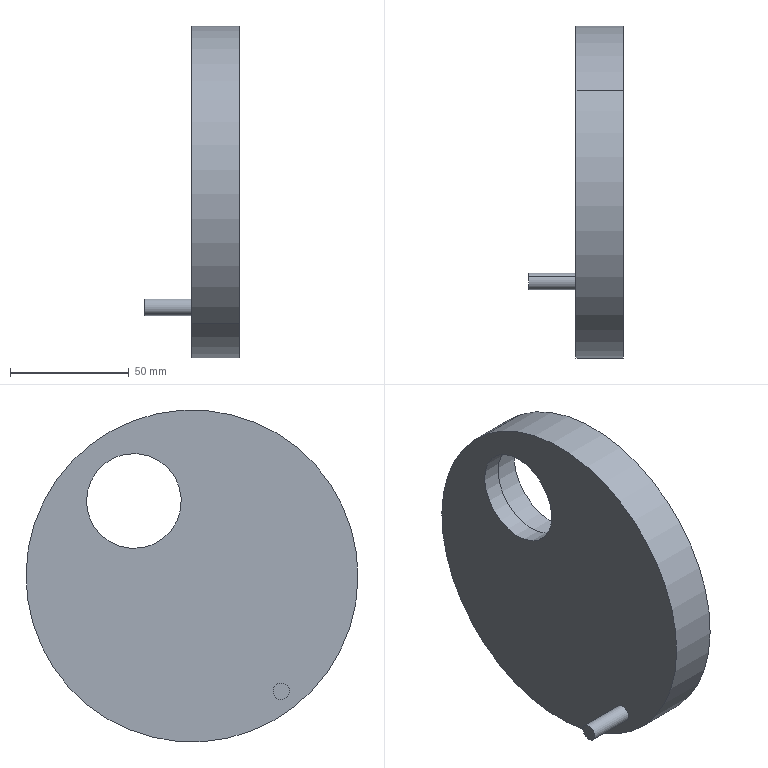Component | SolidWorks | Part1-1 | 1 solid | 12 faces | box 40 x 140 x 140 mm | volume 279507 mm3 | cylinder 8 | plane 4 | commonest cylinder face diameters 45 x2 7 x2 140 x2 40 x2
build123d program:
from build123d import *

# Parameters (mm, degrees)
SKETCH1_2_R          = 70
BOSS_EXTRUDE1_DEPTH  = 20
SKETCH2_R            = 20
CUT_EXTRUDE1_2_DEPTH = 20
SKETCH3_R            = 3.5
BOSS_EXTRUDE2_DEPTH  = 20
SKETCH1_R            = 22.5
CUT_EXTRUDE1_DEPTH   = 12


with BuildPart() as part:
    # Sketch1_2 → Boss-Extrude1 (new body)
    with BuildSketch(Plane(origin=(0, 0, 0), x_dir=(0, 0, -1), z_dir=(1, 0, 0))):
        Circle(SKETCH1_2_R)
    extrude(amount=BOSS_EXTRUDE1_DEPTH)

    # Sketch2 → Cut-Extrude1_2 (cut)
    with BuildSketch(Plane(origin=(20, 0, 0), x_dir=(0, 0, -1), z_dir=(1, 0, 0))):
        with Locations((40, 0)):
            Circle(SKETCH2_R)
    extrude(amount=-CUT_EXTRUDE1_2_DEPTH, mode=Mode.SUBTRACT)

    # Sketch3 → Boss-Extrude2 (add)
    with BuildSketch(Plane(origin=(20, 0, 0), x_dir=(0, 0, -1), z_dir=(1, 0, 0))):
        with Locations((-61.5, 0)):
            Circle(SKETCH3_R)
    extrude(amount=BOSS_EXTRUDE2_DEPTH)

    # Sketch1 → Cut-Extrude1 (cut)
    with BuildSketch(Plane.ZY):
        with Locations((-40, 0)):
            Circle(SKETCH1_R)
    extrude(amount=-CUT_EXTRUDE1_DEPTH, mode=Mode.SUBTRACT)


solid = part.part

# Placed as in the assembly
solid = solid.moved(Location((405.528, -9.187, -141.621), (142.235, 0, -180)))
STEP:
#1=COLOUR_RGB('',0.7922,0.8196,0.9333);
#2=FILL_AREA_STYLE_COLOUR('',#1);
#3=FILL_AREA_STYLE('',(#2));
#4=SURFACE_STYLE_FILL_AREA(#3);
#5=SURFACE_SIDE_STYLE('',(#4));
#6=SURFACE_STYLE_USAGE(.BOTH.,#5);
#7=PRESENTATION_STYLE_ASSIGNMENT((#6));
#8=CARTESIAN_POINT('',(15.493,1.145,-3.63));
#9=VERTEX_POINT('',#8);
#10=CARTESIAN_POINT('',(15.493,0.06026,-5.031));
#11=VERTEX_POINT('',#10);
#12=CARTESIAN_POINT('',(15.493,0.6028,-4.331));
#13=DIRECTION('',(1.,0.,0.));
#14=DIRECTION('',(0.,-0.6124,-0.7905));
#15=AXIS2_PLACEMENT_3D('',#12,#13,#14);
#16=CIRCLE('',#15,0.8858);
#17=EDGE_CURVE('',#9,#11,#16,.T.);
#18=ORIENTED_EDGE('',*,*,#17,.F.);
#19=CARTESIAN_POINT('',(15.966,1.145,-3.63));
#20=VERTEX_POINT('',#19);
#21=CARTESIAN_POINT('',(15.493,1.145,-3.63));
#22=DIRECTION('',(1.,0.,0.));
#23=VECTOR('',#22,39.37);
#24=LINE('',#21,#23);
#25=EDGE_CURVE('',#9,#20,#24,.T.);
#26=ORIENTED_EDGE('',*,*,#25,.T.);
#27=CARTESIAN_POINT('',(15.966,0.06026,-5.031));
#28=VERTEX_POINT('',#27);
#29=CARTESIAN_POINT('',(15.966,0.6028,-4.331));
#30=DIRECTION('',(1.,0.,0.));
#31=DIRECTION('',(0.,-0.6124,-0.7905));
#32=AXIS2_PLACEMENT_3D('',#29,#30,#31);
#33=CIRCLE('',#32,0.8858);
#34=EDGE_CURVE('',#20,#28,#33,.T.);
#35=ORIENTED_EDGE('',*,*,#34,.T.);
#36=CARTESIAN_POINT('',(15.493,0.06026,-5.031));
#37=DIRECTION('',(1.,0.,0.));
#38=VECTOR('',#37,39.37);
#39=LINE('',#36,#38);
#40=EDGE_CURVE('',#11,#28,#39,.T.);
#41=ORIENTED_EDGE('',*,*,#40,.F.);
#42=EDGE_LOOP('',(#18,#26,#35,#41));
#43=FACE_OUTER_BOUND('',#42,.T.);
#44=CARTESIAN_POINT('',(15.493,0.6028,-4.331));
#45=DIRECTION('',(1.,0.,0.));
#46=DIRECTION('',(0.,-0.6124,-0.7905));
#47=AXIS2_PLACEMENT_3D('',#44,#45,#46);
#48=CYLINDRICAL_SURFACE('',#47,0.8858);
#49=ADVANCED_FACE('',(#43),#48,.F.);
#50=CARTESIAN_POINT('',(14.391,-1.76,-7.381));
#51=VERTEX_POINT('',#50);
#52=CARTESIAN_POINT('',(14.391,-1.929,-7.599));
#53=VERTEX_POINT('',#52);
#54=CARTESIAN_POINT('',(14.391,-1.845,-7.49));
#55=DIRECTION('',(-1.,0.,0.));
#56=DIRECTION('',(0.,0.6124,0.7905));
#57=AXIS2_PLACEMENT_3D('',#54,#55,#56);
#58=CIRCLE('',#57,0.1378);
#59=EDGE_CURVE('',#51,#53,#58,.T.);
#60=ORIENTED_EDGE('',*,*,#59,.F.);
#61=CARTESIAN_POINT('',(15.178,-1.76,-7.381));
#62=VERTEX_POINT('',#61);
#63=CARTESIAN_POINT('',(14.391,-1.76,-7.381));
#64=DIRECTION('',(1.,0.,0.));
#65=VECTOR('',#64,39.37);
#66=LINE('',#63,#65);
#67=EDGE_CURVE('',#51,#62,#66,.T.);
#68=ORIENTED_EDGE('',*,*,#67,.T.);
#69=CARTESIAN_POINT('',(15.178,-1.929,-7.599));
#70=VERTEX_POINT('',#69);
#71=CARTESIAN_POINT('',(15.178,-1.845,-7.49));
#72=DIRECTION('',(-1.,0.,0.));
#73=DIRECTION('',(0.,0.6124,0.7905));
#74=AXIS2_PLACEMENT_3D('',#71,#72,#73);
#75=CIRCLE('',#74,0.1378);
#76=EDGE_CURVE('',#62,#70,#75,.T.);
#77=ORIENTED_EDGE('',*,*,#76,.T.);
#78=CARTESIAN_POINT('',(14.391,-1.929,-7.599));
#79=DIRECTION('',(1.,0.,0.));
#80=VECTOR('',#79,39.37);
#81=LINE('',#78,#80);
#82=EDGE_CURVE('',#53,#70,#81,.T.);
#83=ORIENTED_EDGE('',*,*,#82,.F.);
#84=EDGE_LOOP('',(#60,#68,#77,#83));
#85=FACE_OUTER_BOUND('',#84,.T.);
#86=CARTESIAN_POINT('',(14.391,-1.845,-7.49));
#87=DIRECTION('',(1.,0.,0.));
#88=DIRECTION('',(0.,-0.6124,-0.7905));
#89=AXIS2_PLACEMENT_3D('',#86,#87,#88);
#90=CYLINDRICAL_SURFACE('',#89,0.1378);
#91=ADVANCED_FACE('',(#85),#90,.T.);
#92=CARTESIAN_POINT('',(15.178,1.326,-3.397));
#93=VERTEX_POINT('',#92);
#94=CARTESIAN_POINT('',(15.178,-2.049,-7.754));
#95=VERTEX_POINT('',#94);
#96=CARTESIAN_POINT('',(15.178,-0.3617,-5.576));
#97=DIRECTION('',(-1.,0.,0.));
#98=DIRECTION('',(0.,0.6124,0.7905));
#99=AXIS2_PLACEMENT_3D('',#96,#97,#98);
#100=CIRCLE('',#99,2.756);
#101=EDGE_CURVE('',#93,#95,#100,.T.);
#102=ORIENTED_EDGE('',*,*,#101,.F.);
#103=CARTESIAN_POINT('',(15.966,1.326,-3.397));
#104=VERTEX_POINT('',#103);
#105=CARTESIAN_POINT('',(15.178,1.326,-3.397));
#106=DIRECTION('',(1.,0.,0.));
#107=VECTOR('',#106,39.37);
#108=LINE('',#105,#107);
#109=EDGE_CURVE('',#93,#104,#108,.T.);
#110=ORIENTED_EDGE('',*,*,#109,.T.);
#111=CARTESIAN_POINT('',(15.966,-2.049,-7.754));
#112=VERTEX_POINT('',#111);
#113=CARTESIAN_POINT('',(15.966,-0.3617,-5.576));
#114=DIRECTION('',(-1.,0.,0.));
#115=DIRECTION('',(0.,0.6124,0.7905));
#116=AXIS2_PLACEMENT_3D('',#113,#114,#115);
#117=CIRCLE('',#116,2.756);
#118=EDGE_CURVE('',#104,#112,#117,.T.);
#119=ORIENTED_EDGE('',*,*,#118,.T.);
#120=CARTESIAN_POINT('',(15.178,-2.049,-7.754));
#121=DIRECTION('',(1.,0.,0.));
#122=VECTOR('',#121,39.37);
#123=LINE('',#120,#122);
#124=EDGE_CURVE('',#95,#112,#123,.T.);
#125=ORIENTED_EDGE('',*,*,#124,.F.);
#126=EDGE_LOOP('',(#102,#110,#119,#125));
#127=FACE_OUTER_BOUND('',#126,.T.);
#128=CARTESIAN_POINT('',(15.178,-0.3617,-5.576));
#129=DIRECTION('',(1.,0.,0.));
#130=DIRECTION('',(0.,-0.6124,-0.7905));
#131=AXIS2_PLACEMENT_3D('',#128,#129,#130);
#132=CYLINDRICAL_SURFACE('',#131,2.756);
#133=ADVANCED_FACE('',(#127),#132,.T.);
#134=CARTESIAN_POINT('',(15.493,0.1205,-4.953));
#135=VERTEX_POINT('',#134);
#136=CARTESIAN_POINT('',(15.493,1.085,-3.708));
#137=VERTEX_POINT('',#136);
#138=CARTESIAN_POINT('',(15.493,0.6028,-4.331));
#139=DIRECTION('',(-1.,0.,0.));
#140=DIRECTION('',(0.,-0.6124,-0.7905));
#141=AXIS2_PLACEMENT_3D('',#138,#139,#140);
#142=CIRCLE('',#141,0.7874);
#143=EDGE_CURVE('',#135,#137,#142,.T.);
#144=ORIENTED_EDGE('',*,*,#143,.F.);
#145=CARTESIAN_POINT('',(15.178,0.1205,-4.953));
#146=VERTEX_POINT('',#145);
#147=CARTESIAN_POINT('',(15.966,0.1205,-4.953));
#148=DIRECTION('',(-1.,0.,0.));
#149=VECTOR('',#148,39.37);
#150=LINE('',#147,#149);
#151=EDGE_CURVE('',#135,#146,#150,.T.);
#152=ORIENTED_EDGE('',*,*,#151,.T.);
#153=CARTESIAN_POINT('',(15.178,1.085,-3.708));
#154=VERTEX_POINT('',#153);
#155=CARTESIAN_POINT('',(15.178,0.6028,-4.331));
#156=DIRECTION('',(-1.,0.,0.));
#157=DIRECTION('',(0.,0.6124,0.7905));
#158=AXIS2_PLACEMENT_3D('',#155,#156,#157);
#159=CIRCLE('',#158,0.7874);
#160=EDGE_CURVE('',#146,#154,#159,.T.);
#161=ORIENTED_EDGE('',*,*,#160,.T.);
#162=CARTESIAN_POINT('',(15.966,1.085,-3.708));
#163=DIRECTION('',(-1.,0.,0.));
#164=VECTOR('',#163,39.37);
#165=LINE('',#162,#164);
#166=EDGE_CURVE('',#137,#154,#165,.T.);
#167=ORIENTED_EDGE('',*,*,#166,.F.);
#168=EDGE_LOOP('',(#144,#152,#161,#167));
#169=FACE_OUTER_BOUND('',#168,.T.);
#170=CARTESIAN_POINT('',(15.966,0.6028,-4.331));
#171=DIRECTION('',(-1.,0.,0.));
#172=DIRECTION('',(0.,0.6124,0.7905));
#173=AXIS2_PLACEMENT_3D('',#170,#171,#172);
#174=CYLINDRICAL_SURFACE('',#173,0.7874);
#175=ADVANCED_FACE('',(#169),#174,.F.);
#176=ORIENTED_EDGE('',*,*,#151,.F.);
#177=CARTESIAN_POINT('',(15.493,0.6028,-4.331));
#178=DIRECTION('',(-1.,0.,0.));
#179=DIRECTION('',(0.,-0.6124,-0.7905));
#180=AXIS2_PLACEMENT_3D('',#177,#178,#179);
#181=CIRCLE('',#180,0.7874);
#182=EDGE_CURVE('',#137,#135,#181,.T.);
#183=ORIENTED_EDGE('',*,*,#182,.F.);
#184=ORIENTED_EDGE('',*,*,#166,.T.);
#185=CARTESIAN_POINT('',(15.178,0.6028,-4.331));
#186=DIRECTION('',(-1.,0.,0.));
#187=DIRECTION('',(0.,0.6124,0.7905));
#188=AXIS2_PLACEMENT_3D('',#185,#186,#187);
#189=CIRCLE('',#188,0.7874);
#190=EDGE_CURVE('',#154,#146,#189,.T.);
#191=ORIENTED_EDGE('',*,*,#190,.T.);
#192=EDGE_LOOP('',(#176,#183,#184,#191));
#193=FACE_OUTER_BOUND('',#192,.T.);
#194=CARTESIAN_POINT('',(15.966,0.6028,-4.331));
#195=DIRECTION('',(-1.,0.,0.));
#196=DIRECTION('',(0.,0.6124,0.7905));
#197=AXIS2_PLACEMENT_3D('',#194,#195,#196);
#198=CYLINDRICAL_SURFACE('',#197,0.7874);
#199=ADVANCED_FACE('',(#193),#198,.F.);
#200=CARTESIAN_POINT('',(15.178,-0.3617,-5.576));
#201=DIRECTION('',(-1.,0.,0.));
#202=DIRECTION('',(0.,0.6124,0.7905));
#203=AXIS2_PLACEMENT_3D('',#200,#201,#202);
#204=CIRCLE('',#203,2.756);
#205=EDGE_CURVE('',#95,#93,#204,.T.);
#206=ORIENTED_EDGE('',*,*,#205,.T.);
#207=ORIENTED_EDGE('',*,*,#101,.T.);
#208=EDGE_LOOP('',(#206,#207));
#209=FACE_OUTER_BOUND('',#208,.T.);
#210=ORIENTED_EDGE('',*,*,#190,.F.);
#211=ORIENTED_EDGE('',*,*,#160,.F.);
#212=EDGE_LOOP('',(#210,#211));
#213=FACE_BOUND('',#212,.T.);
#214=CARTESIAN_POINT('',(15.178,-1.845,-7.49));
#215=DIRECTION('',(-1.,0.,0.));
#216=DIRECTION('',(0.,0.6124,0.7905));
#217=AXIS2_PLACEMENT_3D('',#214,#215,#216);
#218=CIRCLE('',#217,0.1378);
#219=EDGE_CURVE('',#70,#62,#218,.T.);
#220=ORIENTED_EDGE('',*,*,#219,.F.);
#221=ORIENTED_EDGE('',*,*,#76,.F.);
#222=EDGE_LOOP('',(#220,#221));
#223=FACE_BOUND('',#222,.T.);
#224=CARTESIAN_POINT('',(15.178,-0.3617,-5.576));
#225=DIRECTION('',(-1.,0.,0.));
#226=DIRECTION('',(0.,0.6124,0.7905));
#227=AXIS2_PLACEMENT_3D('',#224,#225,#226);
#228=PLANE('',#227);
#229=ADVANCED_FACE('',(#209,#213,#223),#228,.T.);
#230=ORIENTED_EDGE('',*,*,#109,.F.);
#231=ORIENTED_EDGE('',*,*,#205,.F.);
#232=ORIENTED_EDGE('',*,*,#124,.T.);
#233=CARTESIAN_POINT('',(15.966,-0.3617,-5.576));
#234=DIRECTION('',(-1.,0.,0.));
#235=DIRECTION('',(0.,0.6124,0.7905));
#236=AXIS2_PLACEMENT_3D('',#233,#234,#235);
#237=CIRCLE('',#236,2.756);
#238=EDGE_CURVE('',#112,#104,#237,.T.);
#239=ORIENTED_EDGE('',*,*,#238,.T.);
#240=EDGE_LOOP('',(#230,#231,#232,#239));
#241=FACE_OUTER_BOUND('',#240,.T.);
#242=CARTESIAN_POINT('',(15.178,-0.3617,-5.576));
#243=DIRECTION('',(1.,0.,0.));
#244=DIRECTION('',(0.,-0.6124,-0.7905));
#245=AXIS2_PLACEMENT_3D('',#242,#243,#244);
#246=CYLINDRICAL_SURFACE('',#245,2.756);
#247=ADVANCED_FACE('',(#241),#246,.T.);
#248=CARTESIAN_POINT('',(15.966,0.6028,-4.331));
#249=DIRECTION('',(1.,0.,0.));
#250=DIRECTION('',(0.,-0.6124,-0.7905));
#251=AXIS2_PLACEMENT_3D('',#248,#249,#250);
#252=CIRCLE('',#251,0.8858);
#253=EDGE_CURVE('',#28,#20,#252,.T.);
#254=ORIENTED_EDGE('',*,*,#253,.F.);
#255=ORIENTED_EDGE('',*,*,#34,.F.);
#256=EDGE_LOOP('',(#254,#255));
#257=FACE_BOUND('',#256,.T.);
#258=ORIENTED_EDGE('',*,*,#238,.F.);
#259=ORIENTED_EDGE('',*,*,#118,.F.);
#260=EDGE_LOOP('',(#258,#259));
#261=FACE_OUTER_BOUND('',#260,.T.);
#262=CARTESIAN_POINT('',(15.966,-0.3617,-5.576));
#263=DIRECTION('',(-1.,0.,0.));
#264=DIRECTION('',(0.,0.6124,0.7905));
#265=AXIS2_PLACEMENT_3D('',#262,#263,#264);
#266=PLANE('',#265);
#267=ADVANCED_FACE('',(#257,#261),#266,.F.);
#268=ORIENTED_EDGE('',*,*,#67,.F.);
#269=CARTESIAN_POINT('',(14.391,-1.845,-7.49));
#270=DIRECTION('',(-1.,0.,0.));
#271=DIRECTION('',(0.,0.6124,0.7905));
#272=AXIS2_PLACEMENT_3D('',#269,#270,#271);
#273=CIRCLE('',#272,0.1378);
#274=EDGE_CURVE('',#53,#51,#273,.T.);
#275=ORIENTED_EDGE('',*,*,#274,.F.);
#276=ORIENTED_EDGE('',*,*,#82,.T.);
#277=ORIENTED_EDGE('',*,*,#219,.T.);
#278=EDGE_LOOP('',(#268,#275,#276,#277));
#279=FACE_OUTER_BOUND('',#278,.T.);
#280=CARTESIAN_POINT('',(14.391,-1.845,-7.49));
#281=DIRECTION('',(1.,0.,0.));
#282=DIRECTION('',(0.,-0.6124,-0.7905));
#283=AXIS2_PLACEMENT_3D('',#280,#281,#282);
#284=CYLINDRICAL_SURFACE('',#283,0.1378);
#285=ADVANCED_FACE('',(#279),#284,.T.);
#286=ORIENTED_EDGE('',*,*,#274,.T.);
#287=ORIENTED_EDGE('',*,*,#59,.T.);
#288=EDGE_LOOP('',(#286,#287));
#289=FACE_OUTER_BOUND('',#288,.T.);
#290=CARTESIAN_POINT('',(14.391,-1.845,-7.49));
#291=DIRECTION('',(-1.,0.,0.));
#292=DIRECTION('',(0.,0.6124,0.7905));
#293=AXIS2_PLACEMENT_3D('',#290,#291,#292);
#294=PLANE('',#293);
#295=ADVANCED_FACE('',(#289),#294,.T.);
#296=CARTESIAN_POINT('',(15.493,0.6028,-4.331));
#297=DIRECTION('',(1.,0.,0.));
#298=DIRECTION('',(0.,-0.6124,-0.7905));
#299=AXIS2_PLACEMENT_3D('',#296,#297,#298);
#300=CIRCLE('',#299,0.8858);
#301=EDGE_CURVE('',#11,#9,#300,.T.);
#302=ORIENTED_EDGE('',*,*,#301,.T.);
#303=ORIENTED_EDGE('',*,*,#17,.T.);
#304=EDGE_LOOP('',(#302,#303));
#305=FACE_OUTER_BOUND('',#304,.T.);
#306=ORIENTED_EDGE('',*,*,#182,.T.);
#307=ORIENTED_EDGE('',*,*,#143,.T.);
#308=EDGE_LOOP('',(#306,#307));
#309=FACE_BOUND('',#308,.T.);
#310=CARTESIAN_POINT('',(15.493,0.6028,-4.331));
#311=DIRECTION('',(1.,0.,0.));
#312=DIRECTION('',(0.,-0.6124,-0.7905));
#313=AXIS2_PLACEMENT_3D('',#310,#311,#312);
#314=PLANE('',#313);
#315=ADVANCED_FACE('',(#305,#309),#314,.T.);
#316=ORIENTED_EDGE('',*,*,#25,.F.);
#317=ORIENTED_EDGE('',*,*,#301,.F.);
#318=ORIENTED_EDGE('',*,*,#40,.T.);
#319=ORIENTED_EDGE('',*,*,#253,.T.);
#320=EDGE_LOOP('',(#316,#317,#318,#319));
#321=FACE_OUTER_BOUND('',#320,.T.);
#322=CARTESIAN_POINT('',(15.493,0.6028,-4.331));
#323=DIRECTION('',(1.,0.,0.));
#324=DIRECTION('',(0.,-0.6124,-0.7905));
#325=AXIS2_PLACEMENT_3D('',#322,#323,#324);
#326=CYLINDRICAL_SURFACE('',#325,0.8858);
#327=ADVANCED_FACE('',(#321),#326,.F.);
#328=CLOSED_SHELL('',(#49,#91,#133,#175,#199,#229,#247,#267,#285,#295,#315,#327));
#329=MANIFOLD_SOLID_BREP('',#328);
#330=STYLED_ITEM('',(#7),#329);
#331=(LENGTH_UNIT()NAMED_UNIT(*)SI_UNIT($,.METRE.));
#332=LENGTH_MEASURE_WITH_UNIT(LENGTH_MEASURE(0.0254),#331);
#333=DIMENSIONAL_EXPONENTS(1.,0.,0.,0.,0.,0.,0.);
#334=(CONVERSION_BASED_UNIT('',#332)LENGTH_UNIT()NAMED_UNIT(#333));
#335=UNCERTAINTY_MEASURE_WITH_UNIT(LENGTH_MEASURE(0.00001),#334,'','');
#336=(NAMED_UNIT(*)PLANE_ANGLE_UNIT()SI_UNIT($,.RADIAN.));
#337=(NAMED_UNIT(*)SI_UNIT($,.STERADIAN.)SOLID_ANGLE_UNIT());
#338=(GEOMETRIC_REPRESENTATION_CONTEXT(3)GLOBAL_UNCERTAINTY_ASSIGNED_CONTEXT((#335))GLOBAL_UNIT_ASSIGNED_CONTEXT((#334,#336,#337))REPRESENTATION_CONTEXT('',''));
#339=MECHANICAL_DESIGN_GEOMETRIC_PRESENTATION_REPRESENTATION('',(#330),#338);
#340=CARTESIAN_POINT('',(0.,0.,0.));
#341=DIRECTION('',(0.,0.,1.));
#342=DIRECTION('',(1.,0.,0.));
#343=AXIS2_PLACEMENT_3D('',#340,#341,#342);
#344=(LENGTH_UNIT()NAMED_UNIT(*)SI_UNIT($,.METRE.));
#345=LENGTH_MEASURE_WITH_UNIT(LENGTH_MEASURE(0.0254),#344);
#346=DIMENSIONAL_EXPONENTS(1.,0.,0.,0.,0.,0.,0.);
#347=(CONVERSION_BASED_UNIT('',#345)LENGTH_UNIT()NAMED_UNIT(#346));
#348=UNCERTAINTY_MEASURE_WITH_UNIT(LENGTH_MEASURE(0.00001),#347,'','');
#349=(NAMED_UNIT(*)PLANE_ANGLE_UNIT()SI_UNIT($,.RADIAN.));
#350=(NAMED_UNIT(*)SI_UNIT($,.STERADIAN.)SOLID_ANGLE_UNIT());
#351=(GEOMETRIC_REPRESENTATION_CONTEXT(3)GLOBAL_UNCERTAINTY_ASSIGNED_CONTEXT((#348))GLOBAL_UNIT_ASSIGNED_CONTEXT((#347,#349,#350))REPRESENTATION_CONTEXT('',''));
#352=ADVANCED_BREP_SHAPE_REPRESENTATION('',(#329,#343),#351);
#353=PRESENTATION_LAYER_ASSIGNMENT('','',(#330));